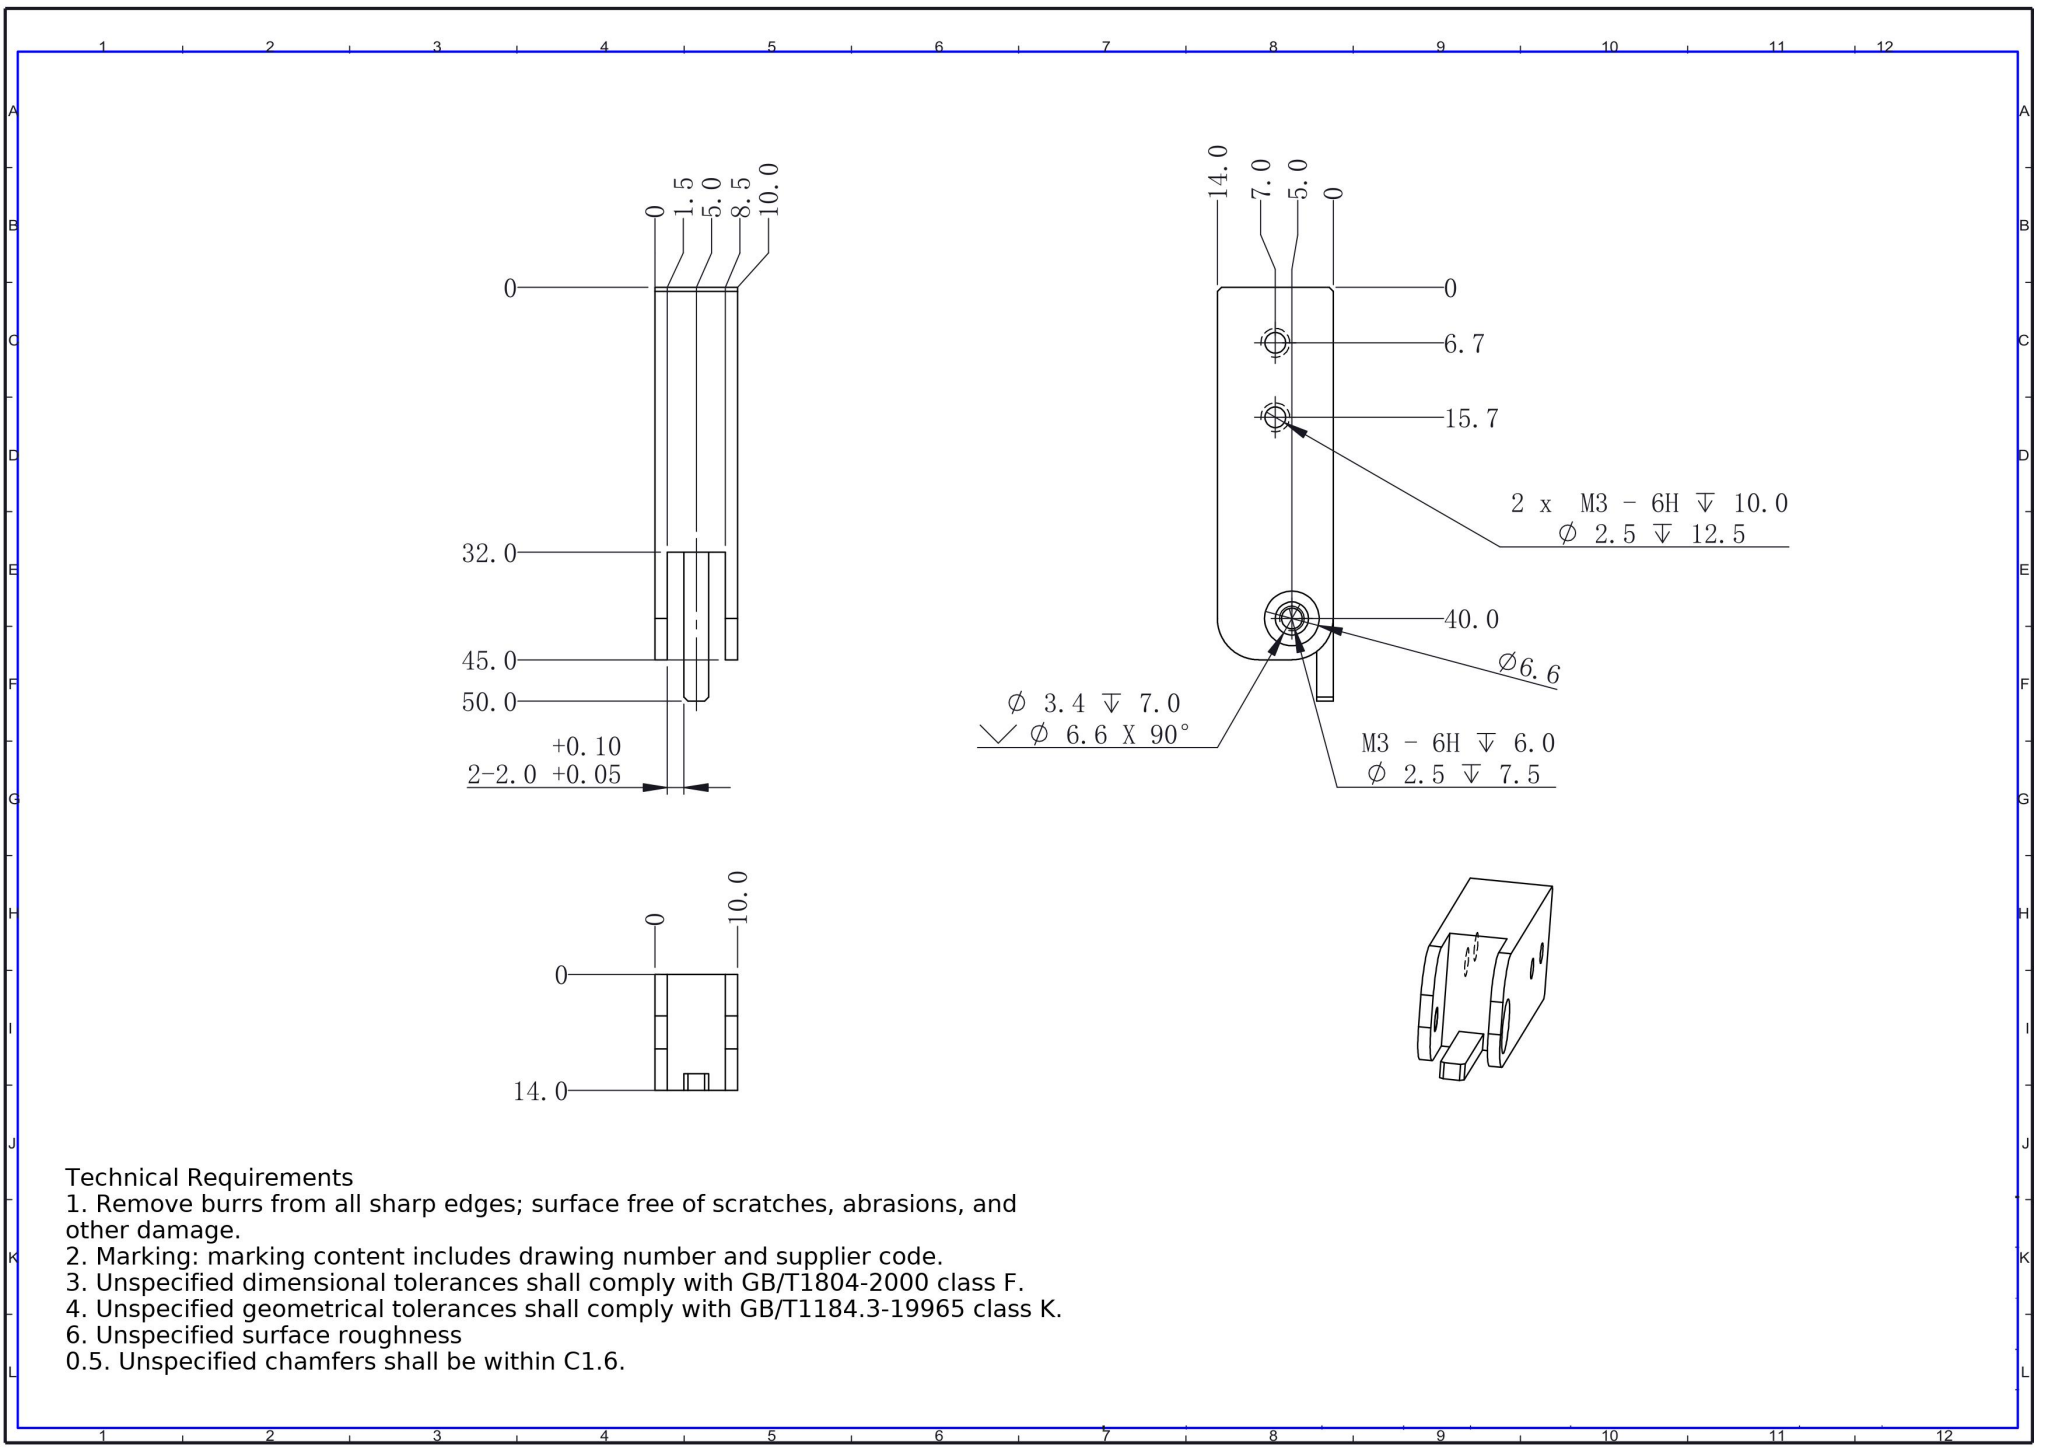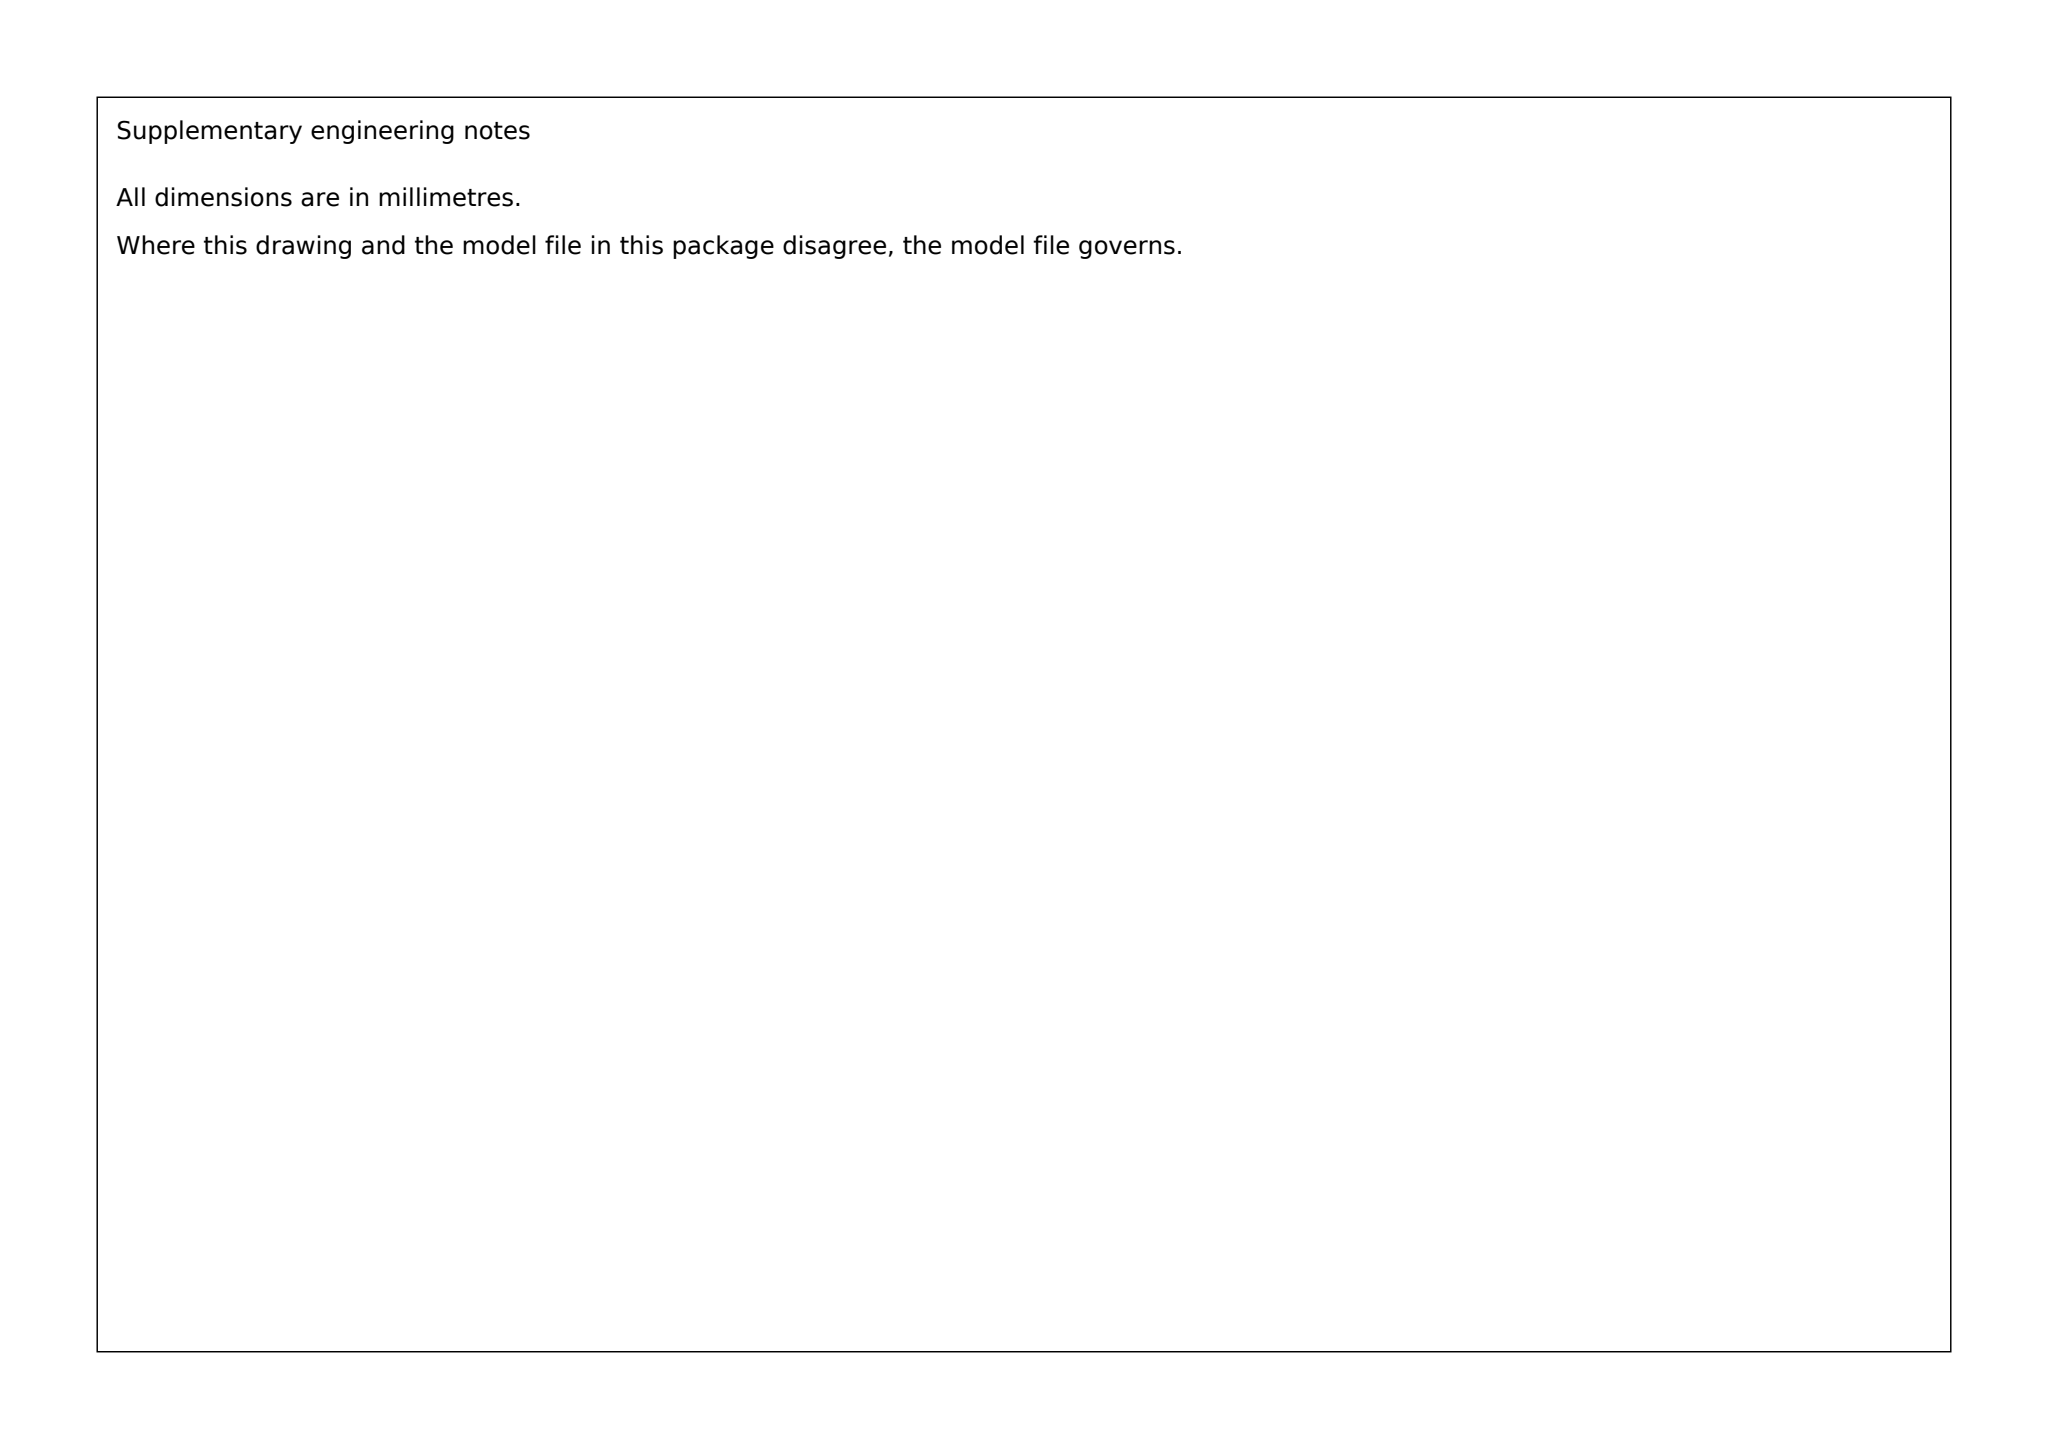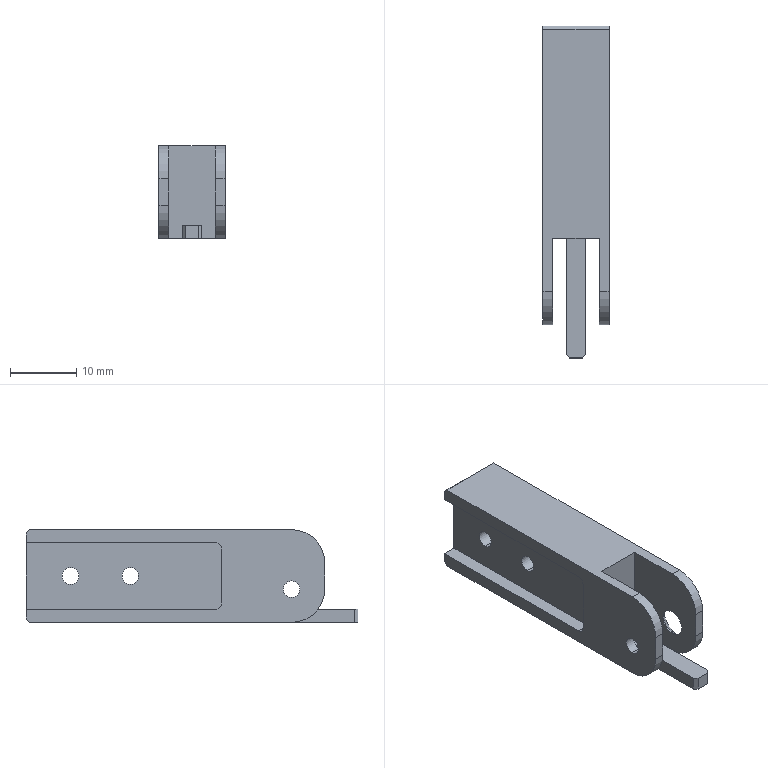Part | SolidWorks | mm | 1 solid | 38 faces | box 10 x 50 x 14 mm | volume 4392 mm3 | plane 22 | cylinder 14 | cone 2 | commonest cylinder face diameters 2.5 x6 10 x4 4 x2 2 x2